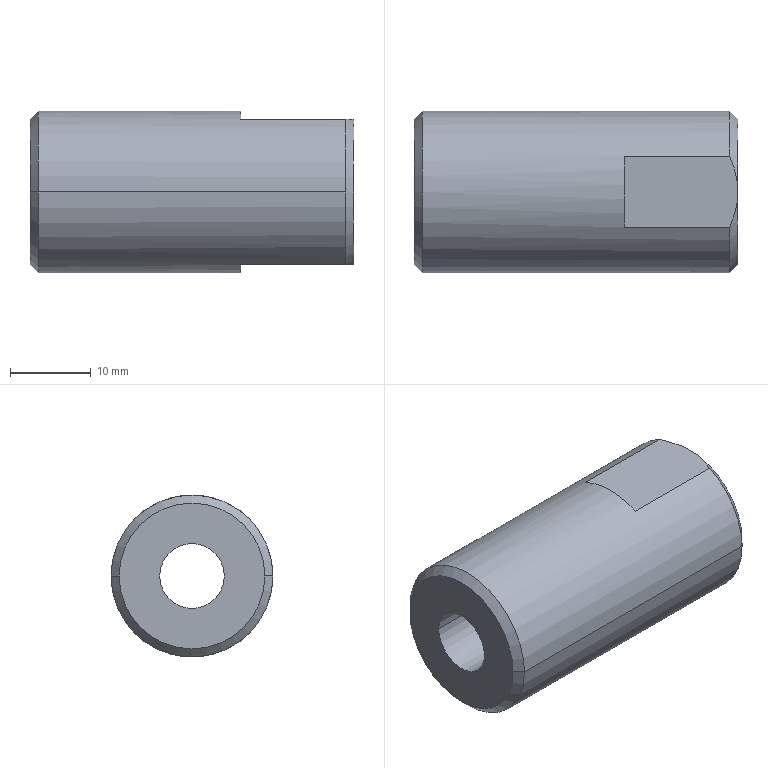Component | SolidWorks | XXXXX08-01-040513-1 | 1 solid | 17 faces | box 40 x 20 x 20 mm | volume 10338 mm3 | cone 7 | plane 6 | cylinder 4 | commonest cylinder face diameters 8 x2 20 x2 | material 45
build123d program:
from build123d import *

# Parameters (mm, degrees)
SKETCH1_R                   = 10
BOSS_EXTRUDE1_DEPTH         = 20
CHAMFER1_SIZE               = 1
M8_TAPPED_HOLE1_D           = 8
M8_TAPPED_HOLE1_CSINK_D     = 8.05
M8_TAPPED_HOLE1_CSINK_ANGLE = 90
CUT_EXTRUDE1_DEPTH          = 25.495
CUT_EXTRUDE1_DEPTH_BACK     = 25.495
SKETCH6_W                   = 14
SKETCH6_H                   = 1


with BuildPart() as part:
    # Sketch1 → Boss-Extrude1 (new, symmetric)
    with BuildSketch(Plane(origin=(0, 0, 0), x_dir=(0, 0, -1), z_dir=(1, 0, 0))):
        Circle(SKETCH1_R)
    extrude(amount=BOSS_EXTRUDE1_DEPTH, both=True)

    # Chamfer1
    chamfer1_edges = [part.edges().sort_by_distance(p)[0] for p in [
        (-20, 0, 10),
        (20, 0, 10),
    ]]
    chamfer(chamfer1_edges, length=CHAMFER1_SIZE)

    # M8 Tapped Hole1 (through all)
    with Locations(Plane.ZY.offset(20)):
        with Locations((0, 0)):
            CounterSinkHole(M8_TAPPED_HOLE1_D / 2, M8_TAPPED_HOLE1_CSINK_D / 2, counter_sink_angle=M8_TAPPED_HOLE1_CSINK_ANGLE)

    # Sketch6 → Cut-Extrude1 (cut, two sides: drawn at the far end of the back side and taken through both)
    with BuildSketch(Plane.XY.offset(-CUT_EXTRUDE1_DEPTH_BACK)):
        with Locations((-13, 9.5)):
            Rectangle(SKETCH6_W, SKETCH6_H)
        with Locations((-13, -9.5)):
            Rectangle(SKETCH6_W, SKETCH6_H)
    extrude(amount=CUT_EXTRUDE1_DEPTH + CUT_EXTRUDE1_DEPTH_BACK, mode=Mode.SUBTRACT)


solid = part.part

# Placed as in the assembly
solid = solid.moved(Location((16, 42.426, 42.426), (-90, 0, 180)))
STEP:
#1=CARTESIAN_POINT('',(1.416,1.828,1.67));
#2=VERTEX_POINT('',#1);
#3=CARTESIAN_POINT('',(1.416,1.513,1.67));
#4=VERTEX_POINT('',#3);
#5=CARTESIAN_POINT('',(1.416,1.67,1.67));
#6=DIRECTION('',(1.,0.,0.));
#7=DIRECTION('',(0.,-1.,0.));
#8=AXIS2_PLACEMENT_3D('',#5,#6,#7);
#9=CIRCLE('',#8,0.1575);
#10=EDGE_CURVE('',#2,#4,#9,.T.);
#11=ORIENTED_EDGE('',*,*,#10,.F.);
#12=CARTESIAN_POINT('',(1.417,1.829,1.67));
#13=VERTEX_POINT('',#12);
#14=CARTESIAN_POINT('',(1.417,1.829,1.67));
#15=DIRECTION('',(0.7071,0.7071,-0.));
#16=VECTOR('',#15,39.37);
#17=LINE('',#14,#16);
#18=EDGE_CURVE('',#2,#13,#17,.T.);
#19=ORIENTED_EDGE('',*,*,#18,.T.);
#20=CARTESIAN_POINT('',(1.417,1.512,1.67));
#21=VERTEX_POINT('',#20);
#22=CARTESIAN_POINT('',(1.417,1.67,1.67));
#23=DIRECTION('',(1.,0.,0.));
#24=DIRECTION('',(0.,-1.,0.));
#25=AXIS2_PLACEMENT_3D('',#22,#23,#24);
#26=CIRCLE('',#25,0.1585);
#27=EDGE_CURVE('',#13,#21,#26,.T.);
#28=ORIENTED_EDGE('',*,*,#27,.T.);
#29=CARTESIAN_POINT('',(1.417,1.512,1.67));
#30=DIRECTION('',(0.7071,-0.7071,0.));
#31=VECTOR('',#30,39.37);
#32=LINE('',#29,#31);
#33=EDGE_CURVE('',#4,#21,#32,.T.);
#34=ORIENTED_EDGE('',*,*,#33,.F.);
#35=EDGE_LOOP('',(#11,#19,#28,#34));
#36=FACE_OUTER_BOUND('',#35,.T.);
#37=CARTESIAN_POINT('',(1.417,1.67,1.67));
#38=DIRECTION('',(1.,0.,0.));
#39=DIRECTION('',(0.,-1.,0.));
#40=AXIS2_PLACEMENT_3D('',#37,#38,#39);
#41=CONICAL_SURFACE('',#40,0.1585,0.7854);
#42=ADVANCED_FACE('',(#36),#41,.F.);
#43=CARTESIAN_POINT('',(-0.1575,1.828,1.67));
#44=VERTEX_POINT('',#43);
#45=CARTESIAN_POINT('',(-0.1575,1.513,1.67));
#46=VERTEX_POINT('',#45);
#47=CARTESIAN_POINT('',(-0.1575,1.67,1.67));
#48=DIRECTION('',(1.,0.,0.));
#49=DIRECTION('',(0.,-1.,0.));
#50=AXIS2_PLACEMENT_3D('',#47,#48,#49);
#51=CIRCLE('',#50,0.1575);
#52=EDGE_CURVE('',#44,#46,#51,.T.);
#53=ORIENTED_EDGE('',*,*,#52,.F.);
#54=CARTESIAN_POINT('',(1.417,1.828,1.67));
#55=DIRECTION('',(1.,0.,0.));
#56=VECTOR('',#55,39.37);
#57=LINE('',#54,#56);
#58=EDGE_CURVE('',#44,#2,#57,.T.);
#59=ORIENTED_EDGE('',*,*,#58,.T.);
#60=ORIENTED_EDGE('',*,*,#10,.T.);
#61=CARTESIAN_POINT('',(1.417,1.513,1.67));
#62=DIRECTION('',(1.,0.,0.));
#63=VECTOR('',#62,39.37);
#64=LINE('',#61,#63);
#65=EDGE_CURVE('',#46,#4,#64,.T.);
#66=ORIENTED_EDGE('',*,*,#65,.F.);
#67=EDGE_LOOP('',(#53,#59,#60,#66));
#68=FACE_OUTER_BOUND('',#67,.T.);
#69=CARTESIAN_POINT('',(1.417,1.67,1.67));
#70=DIRECTION('',(1.,0.,0.));
#71=DIRECTION('',(0.,-1.,0.));
#72=AXIS2_PLACEMENT_3D('',#69,#70,#71);
#73=CYLINDRICAL_SURFACE('',#72,0.1575);
#74=ADVANCED_FACE('',(#68),#73,.F.);
#75=CARTESIAN_POINT('',(1.417,2.025,1.67));
#76=VERTEX_POINT('',#75);
#77=CARTESIAN_POINT('',(1.417,1.67,2.025));
#78=VERTEX_POINT('',#77);
#79=CARTESIAN_POINT('',(1.417,1.67,1.67));
#80=DIRECTION('',(1.,0.,0.));
#81=DIRECTION('',(0.,1.,-0.));
#82=AXIS2_PLACEMENT_3D('',#79,#80,#81);
#83=CIRCLE('',#82,0.3543);
#84=EDGE_CURVE('',#76,#78,#83,.T.);
#85=ORIENTED_EDGE('',*,*,#84,.F.);
#86=CARTESIAN_POINT('',(1.378,2.064,1.67));
#87=VERTEX_POINT('',#86);
#88=CARTESIAN_POINT('',(1.378,2.064,1.67));
#89=DIRECTION('',(-0.7071,0.7071,-0.));
#90=VECTOR('',#89,39.37);
#91=LINE('',#88,#90);
#92=EDGE_CURVE('',#76,#87,#91,.T.);
#93=ORIENTED_EDGE('',*,*,#92,.T.);
#94=CARTESIAN_POINT('',(1.378,1.842,2.025));
#95=VERTEX_POINT('',#94);
#96=CARTESIAN_POINT('',(1.378,1.67,1.67));
#97=DIRECTION('',(-1.,0.,0.));
#98=DIRECTION('',(0.,1.,-0.));
#99=AXIS2_PLACEMENT_3D('',#96,#97,#98);
#100=CIRCLE('',#99,0.3937);
#101=EDGE_CURVE('',#95,#87,#100,.T.);
#102=ORIENTED_EDGE('',*,*,#101,.F.);
#103=CARTESIAN_POINT('',(1.417,1.67,2.025));
#104=CARTESIAN_POINT('',(1.417,1.7,2.025));
#105=CARTESIAN_POINT('',(1.414,1.729,2.025));
#106=CARTESIAN_POINT('',(1.403,1.773,2.025));
#107=CARTESIAN_POINT('',(1.399,1.787,2.025));
#108=CARTESIAN_POINT('',(1.389,1.815,2.025));
#109=CARTESIAN_POINT('',(1.384,1.828,2.025));
#110=CARTESIAN_POINT('',(1.378,1.842,2.025));
#111=B_SPLINE_CURVE_WITH_KNOTS('',3,(#103,#104,#105,#106,#107,#108,#109,#110),.UNSPECIFIED.,.F.,.F.,(4,2,2,4),(0.01099,0.01321,0.01433,0.01544),.UNSPECIFIED.);
#112=EDGE_CURVE('',#78,#95,#111,.T.);
#113=ORIENTED_EDGE('',*,*,#112,.F.);
#114=EDGE_LOOP('',(#85,#93,#102,#113));
#115=FACE_OUTER_BOUND('',#114,.T.);
#116=CARTESIAN_POINT('',(1.378,1.67,1.67));
#117=DIRECTION('',(-1.,0.,0.));
#118=DIRECTION('',(0.,1.,-0.));
#119=AXIS2_PLACEMENT_3D('',#116,#117,#118);
#120=CONICAL_SURFACE('',#119,0.3937,0.7854);
#121=ADVANCED_FACE('',(#115),#120,.T.);
#122=CARTESIAN_POINT('',(-0.1575,2.025,1.67));
#123=VERTEX_POINT('',#122);
#124=CARTESIAN_POINT('',(-0.1575,1.316,1.67));
#125=VERTEX_POINT('',#124);
#126=CARTESIAN_POINT('',(-0.1575,1.67,1.67));
#127=DIRECTION('',(-1.,0.,0.));
#128=DIRECTION('',(0.,1.,-0.));
#129=AXIS2_PLACEMENT_3D('',#126,#127,#128);
#130=CIRCLE('',#129,0.3543);
#131=EDGE_CURVE('',#123,#125,#130,.T.);
#132=ORIENTED_EDGE('',*,*,#131,.F.);
#133=CARTESIAN_POINT('',(-0.1181,2.064,1.67));
#134=VERTEX_POINT('',#133);
#135=CARTESIAN_POINT('',(-0.1575,2.025,1.67));
#136=DIRECTION('',(0.7071,0.7071,-0.));
#137=VECTOR('',#136,39.37);
#138=LINE('',#135,#137);
#139=EDGE_CURVE('',#123,#134,#138,.T.);
#140=ORIENTED_EDGE('',*,*,#139,.T.);
#141=CARTESIAN_POINT('',(-0.1181,1.277,1.67));
#142=VERTEX_POINT('',#141);
#143=CARTESIAN_POINT('',(-0.1181,1.67,1.67));
#144=DIRECTION('',(1.,0.,0.));
#145=DIRECTION('',(0.,1.,-0.));
#146=AXIS2_PLACEMENT_3D('',#143,#144,#145);
#147=CIRCLE('',#146,0.3937);
#148=EDGE_CURVE('',#142,#134,#147,.T.);
#149=ORIENTED_EDGE('',*,*,#148,.F.);
#150=CARTESIAN_POINT('',(-0.1575,1.316,1.67));
#151=DIRECTION('',(0.7071,-0.7071,0.));
#152=VECTOR('',#151,39.37);
#153=LINE('',#150,#152);
#154=EDGE_CURVE('',#125,#142,#153,.T.);
#155=ORIENTED_EDGE('',*,*,#154,.F.);
#156=EDGE_LOOP('',(#132,#140,#149,#155));
#157=FACE_OUTER_BOUND('',#156,.T.);
#158=CARTESIAN_POINT('',(-0.1575,1.67,1.67));
#159=DIRECTION('',(1.,0.,0.));
#160=DIRECTION('',(0.,-1.,0.));
#161=AXIS2_PLACEMENT_3D('',#158,#159,#160);
#162=CONICAL_SURFACE('',#161,0.3543,0.7854);
#163=ADVANCED_FACE('',(#157),#162,.T.);
#164=ORIENTED_EDGE('',*,*,#148,.T.);
#165=CARTESIAN_POINT('',(-0.1575,2.064,1.67));
#166=DIRECTION('',(1.,0.,0.));
#167=VECTOR('',#166,39.37);
#168=LINE('',#165,#167);
#169=EDGE_CURVE('',#134,#87,#168,.T.);
#170=ORIENTED_EDGE('',*,*,#169,.T.);
#171=CARTESIAN_POINT('',(1.378,1.842,1.316));
#172=VERTEX_POINT('',#171);
#173=CARTESIAN_POINT('',(1.378,1.67,1.67));
#174=DIRECTION('',(-1.,0.,0.));
#175=DIRECTION('',(0.,1.,-0.));
#176=AXIS2_PLACEMENT_3D('',#173,#174,#175);
#177=CIRCLE('',#176,0.3937);
#178=EDGE_CURVE('',#87,#172,#177,.T.);
#179=ORIENTED_EDGE('',*,*,#178,.T.);
#180=CARTESIAN_POINT('',(0.8661,1.842,1.316));
#181=VERTEX_POINT('',#180);
#182=CARTESIAN_POINT('',(-0.1575,1.842,1.316));
#183=DIRECTION('',(-1.,0.,0.));
#184=VECTOR('',#183,39.37);
#185=LINE('',#182,#184);
#186=EDGE_CURVE('',#172,#181,#185,.T.);
#187=ORIENTED_EDGE('',*,*,#186,.T.);
#188=CARTESIAN_POINT('',(0.8661,1.499,1.316));
#189=VERTEX_POINT('',#188);
#190=CARTESIAN_POINT('',(0.8661,1.67,1.67));
#191=DIRECTION('',(-1.,0.,0.));
#192=DIRECTION('',(0.,1.,-0.));
#193=AXIS2_PLACEMENT_3D('',#190,#191,#192);
#194=CIRCLE('',#193,0.3937);
#195=EDGE_CURVE('',#181,#189,#194,.T.);
#196=ORIENTED_EDGE('',*,*,#195,.T.);
#197=CARTESIAN_POINT('',(1.378,1.499,1.316));
#198=VERTEX_POINT('',#197);
#199=CARTESIAN_POINT('',(-0.1575,1.499,1.316));
#200=DIRECTION('',(1.,0.,0.));
#201=VECTOR('',#200,39.37);
#202=LINE('',#199,#201);
#203=EDGE_CURVE('',#189,#198,#202,.T.);
#204=ORIENTED_EDGE('',*,*,#203,.T.);
#205=CARTESIAN_POINT('',(1.378,1.277,1.67));
#206=VERTEX_POINT('',#205);
#207=CARTESIAN_POINT('',(1.378,1.67,1.67));
#208=DIRECTION('',(-1.,0.,0.));
#209=DIRECTION('',(0.,1.,-0.));
#210=AXIS2_PLACEMENT_3D('',#207,#208,#209);
#211=CIRCLE('',#210,0.3937);
#212=EDGE_CURVE('',#198,#206,#211,.T.);
#213=ORIENTED_EDGE('',*,*,#212,.T.);
#214=CARTESIAN_POINT('',(-0.1575,1.277,1.67));
#215=DIRECTION('',(1.,0.,0.));
#216=VECTOR('',#215,39.37);
#217=LINE('',#214,#216);
#218=EDGE_CURVE('',#142,#206,#217,.T.);
#219=ORIENTED_EDGE('',*,*,#218,.F.);
#220=EDGE_LOOP('',(#164,#170,#179,#187,#196,#204,#213,#219));
#221=FACE_OUTER_BOUND('',#220,.T.);
#222=CARTESIAN_POINT('',(-0.1575,1.67,1.67));
#223=DIRECTION('',(1.,0.,0.));
#224=DIRECTION('',(0.,-1.,0.));
#225=AXIS2_PLACEMENT_3D('',#222,#223,#224);
#226=CYLINDRICAL_SURFACE('',#225,0.3937);
#227=ADVANCED_FACE('',(#221),#226,.T.);
#228=CARTESIAN_POINT('',(1.378,1.499,2.025));
#229=VERTEX_POINT('',#228);
#230=CARTESIAN_POINT('',(1.378,1.499,2.025));
#231=CARTESIAN_POINT('',(1.39,1.526,2.025));
#232=CARTESIAN_POINT('',(1.4,1.554,2.025));
#233=CARTESIAN_POINT('',(1.41,1.597,2.025));
#234=CARTESIAN_POINT('',(1.413,1.611,2.025));
#235=CARTESIAN_POINT('',(1.416,1.641,2.025));
#236=CARTESIAN_POINT('',(1.417,1.655,2.025));
#237=CARTESIAN_POINT('',(1.417,1.67,2.025));
#238=B_SPLINE_CURVE_WITH_KNOTS('',3,(#230,#231,#232,#233,#234,#235,#236,#237),.UNSPECIFIED.,.F.,.F.,(4,2,2,4),(0.006532,0.008759,0.009873,0.01099),.UNSPECIFIED.);
#239=EDGE_CURVE('',#229,#78,#238,.T.);
#240=ORIENTED_EDGE('',*,*,#239,.F.);
#241=CARTESIAN_POINT('',(1.378,1.67,1.67));
#242=DIRECTION('',(-1.,0.,0.));
#243=DIRECTION('',(0.,1.,-0.));
#244=AXIS2_PLACEMENT_3D('',#241,#242,#243);
#245=CIRCLE('',#244,0.3937);
#246=EDGE_CURVE('',#206,#229,#245,.T.);
#247=ORIENTED_EDGE('',*,*,#246,.F.);
#248=ORIENTED_EDGE('',*,*,#212,.F.);
#249=CARTESIAN_POINT('',(1.417,1.67,1.316));
#250=VERTEX_POINT('',#249);
#251=CARTESIAN_POINT('',(1.417,1.67,1.316));
#252=CARTESIAN_POINT('',(1.417,1.655,1.316));
#253=CARTESIAN_POINT('',(1.416,1.641,1.316));
#254=CARTESIAN_POINT('',(1.413,1.611,1.316));
#255=CARTESIAN_POINT('',(1.41,1.597,1.316));
#256=CARTESIAN_POINT('',(1.4,1.554,1.316));
#257=CARTESIAN_POINT('',(1.39,1.526,1.316));
#258=CARTESIAN_POINT('',(1.378,1.499,1.316));
#259=B_SPLINE_CURVE_WITH_KNOTS('',3,(#251,#252,#253,#254,#255,#256,#257,#258),.UNSPECIFIED.,.F.,.F.,(4,2,2,4),(0.007338,0.008458,0.009578,0.01182),.UNSPECIFIED.);
#260=EDGE_CURVE('',#250,#198,#259,.T.);
#261=ORIENTED_EDGE('',*,*,#260,.F.);
#262=CARTESIAN_POINT('',(1.417,1.67,1.67));
#263=DIRECTION('',(1.,0.,0.));
#264=DIRECTION('',(0.,1.,-0.));
#265=AXIS2_PLACEMENT_3D('',#262,#263,#264);
#266=CIRCLE('',#265,0.3543);
#267=EDGE_CURVE('',#78,#250,#266,.T.);
#268=ORIENTED_EDGE('',*,*,#267,.F.);
#269=EDGE_LOOP('',(#240,#247,#248,#261,#268));
#270=FACE_OUTER_BOUND('',#269,.T.);
#271=CARTESIAN_POINT('',(1.378,1.67,1.67));
#272=DIRECTION('',(-1.,0.,0.));
#273=DIRECTION('',(0.,1.,-0.));
#274=AXIS2_PLACEMENT_3D('',#271,#272,#273);
#275=CONICAL_SURFACE('',#274,0.3937,0.7854);
#276=ADVANCED_FACE('',(#270),#275,.T.);
#277=ORIENTED_EDGE('',*,*,#169,.F.);
#278=CARTESIAN_POINT('',(-0.1181,1.67,1.67));
#279=DIRECTION('',(1.,0.,0.));
#280=DIRECTION('',(0.,1.,-0.));
#281=AXIS2_PLACEMENT_3D('',#278,#279,#280);
#282=CIRCLE('',#281,0.3937);
#283=EDGE_CURVE('',#134,#142,#282,.T.);
#284=ORIENTED_EDGE('',*,*,#283,.T.);
#285=ORIENTED_EDGE('',*,*,#218,.T.);
#286=ORIENTED_EDGE('',*,*,#246,.T.);
#287=CARTESIAN_POINT('',(0.8661,1.499,2.025));
#288=VERTEX_POINT('',#287);
#289=CARTESIAN_POINT('',(-0.1575,1.499,2.025));
#290=DIRECTION('',(-1.,0.,0.));
#291=VECTOR('',#290,39.37);
#292=LINE('',#289,#291);
#293=EDGE_CURVE('',#229,#288,#292,.T.);
#294=ORIENTED_EDGE('',*,*,#293,.T.);
#295=CARTESIAN_POINT('',(0.8661,1.842,2.025));
#296=VERTEX_POINT('',#295);
#297=CARTESIAN_POINT('',(0.8661,1.67,1.67));
#298=DIRECTION('',(-1.,0.,0.));
#299=DIRECTION('',(0.,1.,-0.));
#300=AXIS2_PLACEMENT_3D('',#297,#298,#299);
#301=CIRCLE('',#300,0.3937);
#302=EDGE_CURVE('',#288,#296,#301,.T.);
#303=ORIENTED_EDGE('',*,*,#302,.T.);
#304=CARTESIAN_POINT('',(-0.1575,1.842,2.025));
#305=DIRECTION('',(1.,0.,0.));
#306=VECTOR('',#305,39.37);
#307=LINE('',#304,#306);
#308=EDGE_CURVE('',#296,#95,#307,.T.);
#309=ORIENTED_EDGE('',*,*,#308,.T.);
#310=ORIENTED_EDGE('',*,*,#101,.T.);
#311=EDGE_LOOP('',(#277,#284,#285,#286,#294,#303,#309,#310));
#312=FACE_OUTER_BOUND('',#311,.T.);
#313=CARTESIAN_POINT('',(-0.1575,1.67,1.67));
#314=DIRECTION('',(1.,0.,0.));
#315=DIRECTION('',(0.,-1.,0.));
#316=AXIS2_PLACEMENT_3D('',#313,#314,#315);
#317=CYLINDRICAL_SURFACE('',#316,0.3937);
#318=ADVANCED_FACE('',(#312),#317,.T.);
#319=CARTESIAN_POINT('',(-0.1575,1.67,1.67));
#320=DIRECTION('',(1.,0.,0.));
#321=DIRECTION('',(0.,-1.,0.));
#322=AXIS2_PLACEMENT_3D('',#319,#320,#321);
#323=CIRCLE('',#322,0.1575);
#324=EDGE_CURVE('',#46,#44,#323,.T.);
#325=ORIENTED_EDGE('',*,*,#324,.T.);
#326=ORIENTED_EDGE('',*,*,#52,.T.);
#327=EDGE_LOOP('',(#325,#326));
#328=FACE_BOUND('',#327,.T.);
#329=CARTESIAN_POINT('',(-0.1575,1.67,1.67));
#330=DIRECTION('',(-1.,0.,0.));
#331=DIRECTION('',(0.,1.,-0.));
#332=AXIS2_PLACEMENT_3D('',#329,#330,#331);
#333=CIRCLE('',#332,0.3543);
#334=EDGE_CURVE('',#125,#123,#333,.T.);
#335=ORIENTED_EDGE('',*,*,#334,.T.);
#336=ORIENTED_EDGE('',*,*,#131,.T.);
#337=EDGE_LOOP('',(#335,#336));
#338=FACE_OUTER_BOUND('',#337,.T.);
#339=CARTESIAN_POINT('',(-0.1575,1.67,1.67));
#340=DIRECTION('',(-1.,0.,0.));
#341=DIRECTION('',(0.,1.,-0.));
#342=AXIS2_PLACEMENT_3D('',#339,#340,#341);
#343=PLANE('',#342);
#344=ADVANCED_FACE('',(#328,#338),#343,.T.);
#345=CARTESIAN_POINT('',(1.417,1.67,1.67));
#346=DIRECTION('',(1.,0.,0.));
#347=DIRECTION('',(0.,-1.,0.));
#348=AXIS2_PLACEMENT_3D('',#345,#346,#347);
#349=CIRCLE('',#348,0.1585);
#350=EDGE_CURVE('',#21,#13,#349,.T.);
#351=ORIENTED_EDGE('',*,*,#350,.F.);
#352=ORIENTED_EDGE('',*,*,#27,.F.);
#353=EDGE_LOOP('',(#351,#352));
#354=FACE_BOUND('',#353,.T.);
#355=CARTESIAN_POINT('',(1.417,1.67,1.67));
#356=DIRECTION('',(1.,0.,0.));
#357=DIRECTION('',(0.,1.,-0.));
#358=AXIS2_PLACEMENT_3D('',#355,#356,#357);
#359=CIRCLE('',#358,0.3543);
#360=EDGE_CURVE('',#250,#76,#359,.T.);
#361=ORIENTED_EDGE('',*,*,#360,.T.);
#362=ORIENTED_EDGE('',*,*,#84,.T.);
#363=ORIENTED_EDGE('',*,*,#267,.T.);
#364=EDGE_LOOP('',(#361,#362,#363));
#365=FACE_OUTER_BOUND('',#364,.T.);
#366=CARTESIAN_POINT('',(1.417,1.67,1.67));
#367=DIRECTION('',(-1.,0.,0.));
#368=DIRECTION('',(0.,1.,-0.));
#369=AXIS2_PLACEMENT_3D('',#366,#367,#368);
#370=PLANE('',#369);
#371=ADVANCED_FACE('',(#354,#365),#370,.F.);
#372=ORIENTED_EDGE('',*,*,#139,.F.);
#373=ORIENTED_EDGE('',*,*,#334,.F.);
#374=ORIENTED_EDGE('',*,*,#154,.T.);
#375=ORIENTED_EDGE('',*,*,#283,.F.);
#376=EDGE_LOOP('',(#372,#373,#374,#375));
#377=FACE_OUTER_BOUND('',#376,.T.);
#378=CARTESIAN_POINT('',(-0.1575,1.67,1.67));
#379=DIRECTION('',(1.,0.,0.));
#380=DIRECTION('',(0.,-1.,0.));
#381=AXIS2_PLACEMENT_3D('',#378,#379,#380);
#382=CONICAL_SURFACE('',#381,0.3543,0.7854);
#383=ADVANCED_FACE('',(#377),#382,.T.);
#384=ORIENTED_EDGE('',*,*,#92,.F.);
#385=ORIENTED_EDGE('',*,*,#360,.F.);
#386=CARTESIAN_POINT('',(1.378,1.842,1.316));
#387=CARTESIAN_POINT('',(1.384,1.828,1.316));
#388=CARTESIAN_POINT('',(1.389,1.815,1.316));
#389=CARTESIAN_POINT('',(1.399,1.787,1.316));
#390=CARTESIAN_POINT('',(1.403,1.773,1.316));
#391=CARTESIAN_POINT('',(1.414,1.729,1.316));
#392=CARTESIAN_POINT('',(1.417,1.7,1.316));
#393=CARTESIAN_POINT('',(1.417,1.67,1.316));
#394=B_SPLINE_CURVE_WITH_KNOTS('',3,(#386,#387,#388,#389,#390,#391,#392,#393),.UNSPECIFIED.,.F.,.F.,(4,2,2,4),(0.002859,0.003979,0.005098,0.007338),.UNSPECIFIED.);
#395=EDGE_CURVE('',#172,#250,#394,.T.);
#396=ORIENTED_EDGE('',*,*,#395,.F.);
#397=ORIENTED_EDGE('',*,*,#178,.F.);
#398=EDGE_LOOP('',(#384,#385,#396,#397));
#399=FACE_OUTER_BOUND('',#398,.T.);
#400=CARTESIAN_POINT('',(1.378,1.67,1.67));
#401=DIRECTION('',(-1.,0.,0.));
#402=DIRECTION('',(0.,1.,-0.));
#403=AXIS2_PLACEMENT_3D('',#400,#401,#402);
#404=CONICAL_SURFACE('',#403,0.3937,0.7854);
#405=ADVANCED_FACE('',(#399),#404,.T.);
#406=ORIENTED_EDGE('',*,*,#58,.F.);
#407=ORIENTED_EDGE('',*,*,#324,.F.);
#408=ORIENTED_EDGE('',*,*,#65,.T.);
#409=CARTESIAN_POINT('',(1.416,1.67,1.67));
#410=DIRECTION('',(1.,0.,0.));
#411=DIRECTION('',(0.,-1.,0.));
#412=AXIS2_PLACEMENT_3D('',#409,#410,#411);
#413=CIRCLE('',#412,0.1575);
#414=EDGE_CURVE('',#4,#2,#413,.T.);
#415=ORIENTED_EDGE('',*,*,#414,.T.);
#416=EDGE_LOOP('',(#406,#407,#408,#415));
#417=FACE_OUTER_BOUND('',#416,.T.);
#418=CARTESIAN_POINT('',(1.417,1.67,1.67));
#419=DIRECTION('',(1.,0.,0.));
#420=DIRECTION('',(0.,-1.,0.));
#421=AXIS2_PLACEMENT_3D('',#418,#419,#420);
#422=CYLINDRICAL_SURFACE('',#421,0.1575);
#423=ADVANCED_FACE('',(#417),#422,.F.);
#424=ORIENTED_EDGE('',*,*,#18,.F.);
#425=ORIENTED_EDGE('',*,*,#414,.F.);
#426=ORIENTED_EDGE('',*,*,#33,.T.);
#427=ORIENTED_EDGE('',*,*,#350,.T.);
#428=EDGE_LOOP('',(#424,#425,#426,#427));
#429=FACE_OUTER_BOUND('',#428,.T.);
#430=CARTESIAN_POINT('',(1.417,1.67,1.67));
#431=DIRECTION('',(1.,0.,0.));
#432=DIRECTION('',(0.,-1.,0.));
#433=AXIS2_PLACEMENT_3D('',#430,#431,#432);
#434=CONICAL_SURFACE('',#433,0.1585,0.7854);
#435=ADVANCED_FACE('',(#429),#434,.F.);
#436=CARTESIAN_POINT('',(0.8661,2.064,1.316));
#437=DIRECTION('',(0.,-1.,0.));
#438=VECTOR('',#437,39.37);
#439=LINE('',#436,#438);
#440=EDGE_CURVE('',#181,#189,#439,.T.);
#441=ORIENTED_EDGE('',*,*,#440,.T.);
#442=ORIENTED_EDGE('',*,*,#195,.F.);
#443=EDGE_LOOP('',(#441,#442));
#444=FACE_OUTER_BOUND('',#443,.T.);
#445=CARTESIAN_POINT('',(0.8661,2.064,1.316));
#446=DIRECTION('',(-1.,0.,0.));
#447=DIRECTION('',(0.,1.,-0.));
#448=AXIS2_PLACEMENT_3D('',#445,#446,#447);
#449=PLANE('',#448);
#450=ADVANCED_FACE('',(#444),#449,.F.);
#451=ORIENTED_EDGE('',*,*,#440,.F.);
#452=ORIENTED_EDGE('',*,*,#186,.F.);
#453=ORIENTED_EDGE('',*,*,#395,.T.);
#454=ORIENTED_EDGE('',*,*,#260,.T.);
#455=ORIENTED_EDGE('',*,*,#203,.F.);
#456=EDGE_LOOP('',(#451,#452,#453,#454,#455));
#457=FACE_OUTER_BOUND('',#456,.T.);
#458=CARTESIAN_POINT('',(1.417,2.064,1.316));
#459=DIRECTION('',(0.,0.,1.));
#460=DIRECTION('',(0.,1.,-0.));
#461=AXIS2_PLACEMENT_3D('',#458,#459,#460);
#462=PLANE('',#461);
#463=ADVANCED_FACE('',(#457),#462,.F.);
#464=CARTESIAN_POINT('',(0.8661,2.064,2.025));
#465=DIRECTION('',(0.,-1.,0.));
#466=VECTOR('',#465,39.37);
#467=LINE('',#464,#466);
#468=EDGE_CURVE('',#296,#288,#467,.T.);
#469=ORIENTED_EDGE('',*,*,#468,.F.);
#470=ORIENTED_EDGE('',*,*,#302,.F.);
#471=EDGE_LOOP('',(#469,#470));
#472=FACE_OUTER_BOUND('',#471,.T.);
#473=CARTESIAN_POINT('',(0.8661,2.064,2.025));
#474=DIRECTION('',(-1.,0.,0.));
#475=DIRECTION('',(0.,1.,-0.));
#476=AXIS2_PLACEMENT_3D('',#473,#474,#475);
#477=PLANE('',#476);
#478=ADVANCED_FACE('',(#472),#477,.F.);
#479=ORIENTED_EDGE('',*,*,#468,.T.);
#480=ORIENTED_EDGE('',*,*,#293,.F.);
#481=ORIENTED_EDGE('',*,*,#239,.T.);
#482=ORIENTED_EDGE('',*,*,#112,.T.);
#483=ORIENTED_EDGE('',*,*,#308,.F.);
#484=EDGE_LOOP('',(#479,#480,#481,#482,#483));
#485=FACE_OUTER_BOUND('',#484,.T.);
#486=CARTESIAN_POINT('',(1.417,2.064,2.025));
#487=DIRECTION('',(0.,-0.,-1.));
#488=DIRECTION('',(0.,-1.,0.));
#489=AXIS2_PLACEMENT_3D('',#486,#487,#488);
#490=PLANE('',#489);
#491=ADVANCED_FACE('',(#485),#490,.F.);
#492=CLOSED_SHELL('',(#42,#74,#121,#163,#227,#276,#318,#344,#371,#383,#405,#423,#435,#450,#463,#478,#491));
#493=MANIFOLD_SOLID_BREP('',#492);
#494=CARTESIAN_POINT('',(0.,0.,0.));
#495=DIRECTION('',(0.,0.,1.));
#496=DIRECTION('',(1.,0.,0.));
#497=AXIS2_PLACEMENT_3D('',#494,#495,#496);
#498=(LENGTH_UNIT()NAMED_UNIT(*)SI_UNIT($,.METRE.));
#499=LENGTH_MEASURE_WITH_UNIT(LENGTH_MEASURE(0.0254),#498);
#500=DIMENSIONAL_EXPONENTS(1.,0.,0.,0.,0.,0.,0.);
#501=(CONVERSION_BASED_UNIT('',#499)LENGTH_UNIT()NAMED_UNIT(#500));
#502=UNCERTAINTY_MEASURE_WITH_UNIT(LENGTH_MEASURE(0.00001),#501,'','');
#503=(NAMED_UNIT(*)PLANE_ANGLE_UNIT()SI_UNIT($,.RADIAN.));
#504=(NAMED_UNIT(*)SI_UNIT($,.STERADIAN.)SOLID_ANGLE_UNIT());
#505=(GEOMETRIC_REPRESENTATION_CONTEXT(3)GLOBAL_UNCERTAINTY_ASSIGNED_CONTEXT((#502))GLOBAL_UNIT_ASSIGNED_CONTEXT((#501,#503,#504))REPRESENTATION_CONTEXT('',''));
#506=ADVANCED_BREP_SHAPE_REPRESENTATION('',(#493,#497),#505);
#507=COLOUR_RGB('',0.7922,0.8196,0.9333);
#508=FILL_AREA_STYLE_COLOUR('',#507);
#509=FILL_AREA_STYLE('',(#508));
#510=SURFACE_STYLE_FILL_AREA(#509);
#511=SURFACE_SIDE_STYLE('',(#510));
#512=SURFACE_STYLE_USAGE(.BOTH.,#511);
#513=PRESENTATION_STYLE_ASSIGNMENT((#512));
#514=STYLED_ITEM('',(#513),#493);
#515=PRESENTATION_LAYER_ASSIGNMENT('','',(#514));
#516=(LENGTH_UNIT()NAMED_UNIT(*)SI_UNIT($,.METRE.));
#517=LENGTH_MEASURE_WITH_UNIT(LENGTH_MEASURE(0.0254),#516);
#518=DIMENSIONAL_EXPONENTS(1.,0.,0.,0.,0.,0.,0.);
#519=(CONVERSION_BASED_UNIT('',#517)LENGTH_UNIT()NAMED_UNIT(#518));
#520=UNCERTAINTY_MEASURE_WITH_UNIT(LENGTH_MEASURE(0.00001),#519,'','');
#521=(NAMED_UNIT(*)PLANE_ANGLE_UNIT()SI_UNIT($,.RADIAN.));
#522=(NAMED_UNIT(*)SI_UNIT($,.STERADIAN.)SOLID_ANGLE_UNIT());
#523=(GEOMETRIC_REPRESENTATION_CONTEXT(3)GLOBAL_UNCERTAINTY_ASSIGNED_CONTEXT((#520))GLOBAL_UNIT_ASSIGNED_CONTEXT((#519,#521,#522))REPRESENTATION_CONTEXT('',''));
#524=MECHANICAL_DESIGN_GEOMETRIC_PRESENTATION_REPRESENTATION('',(#514),#523);